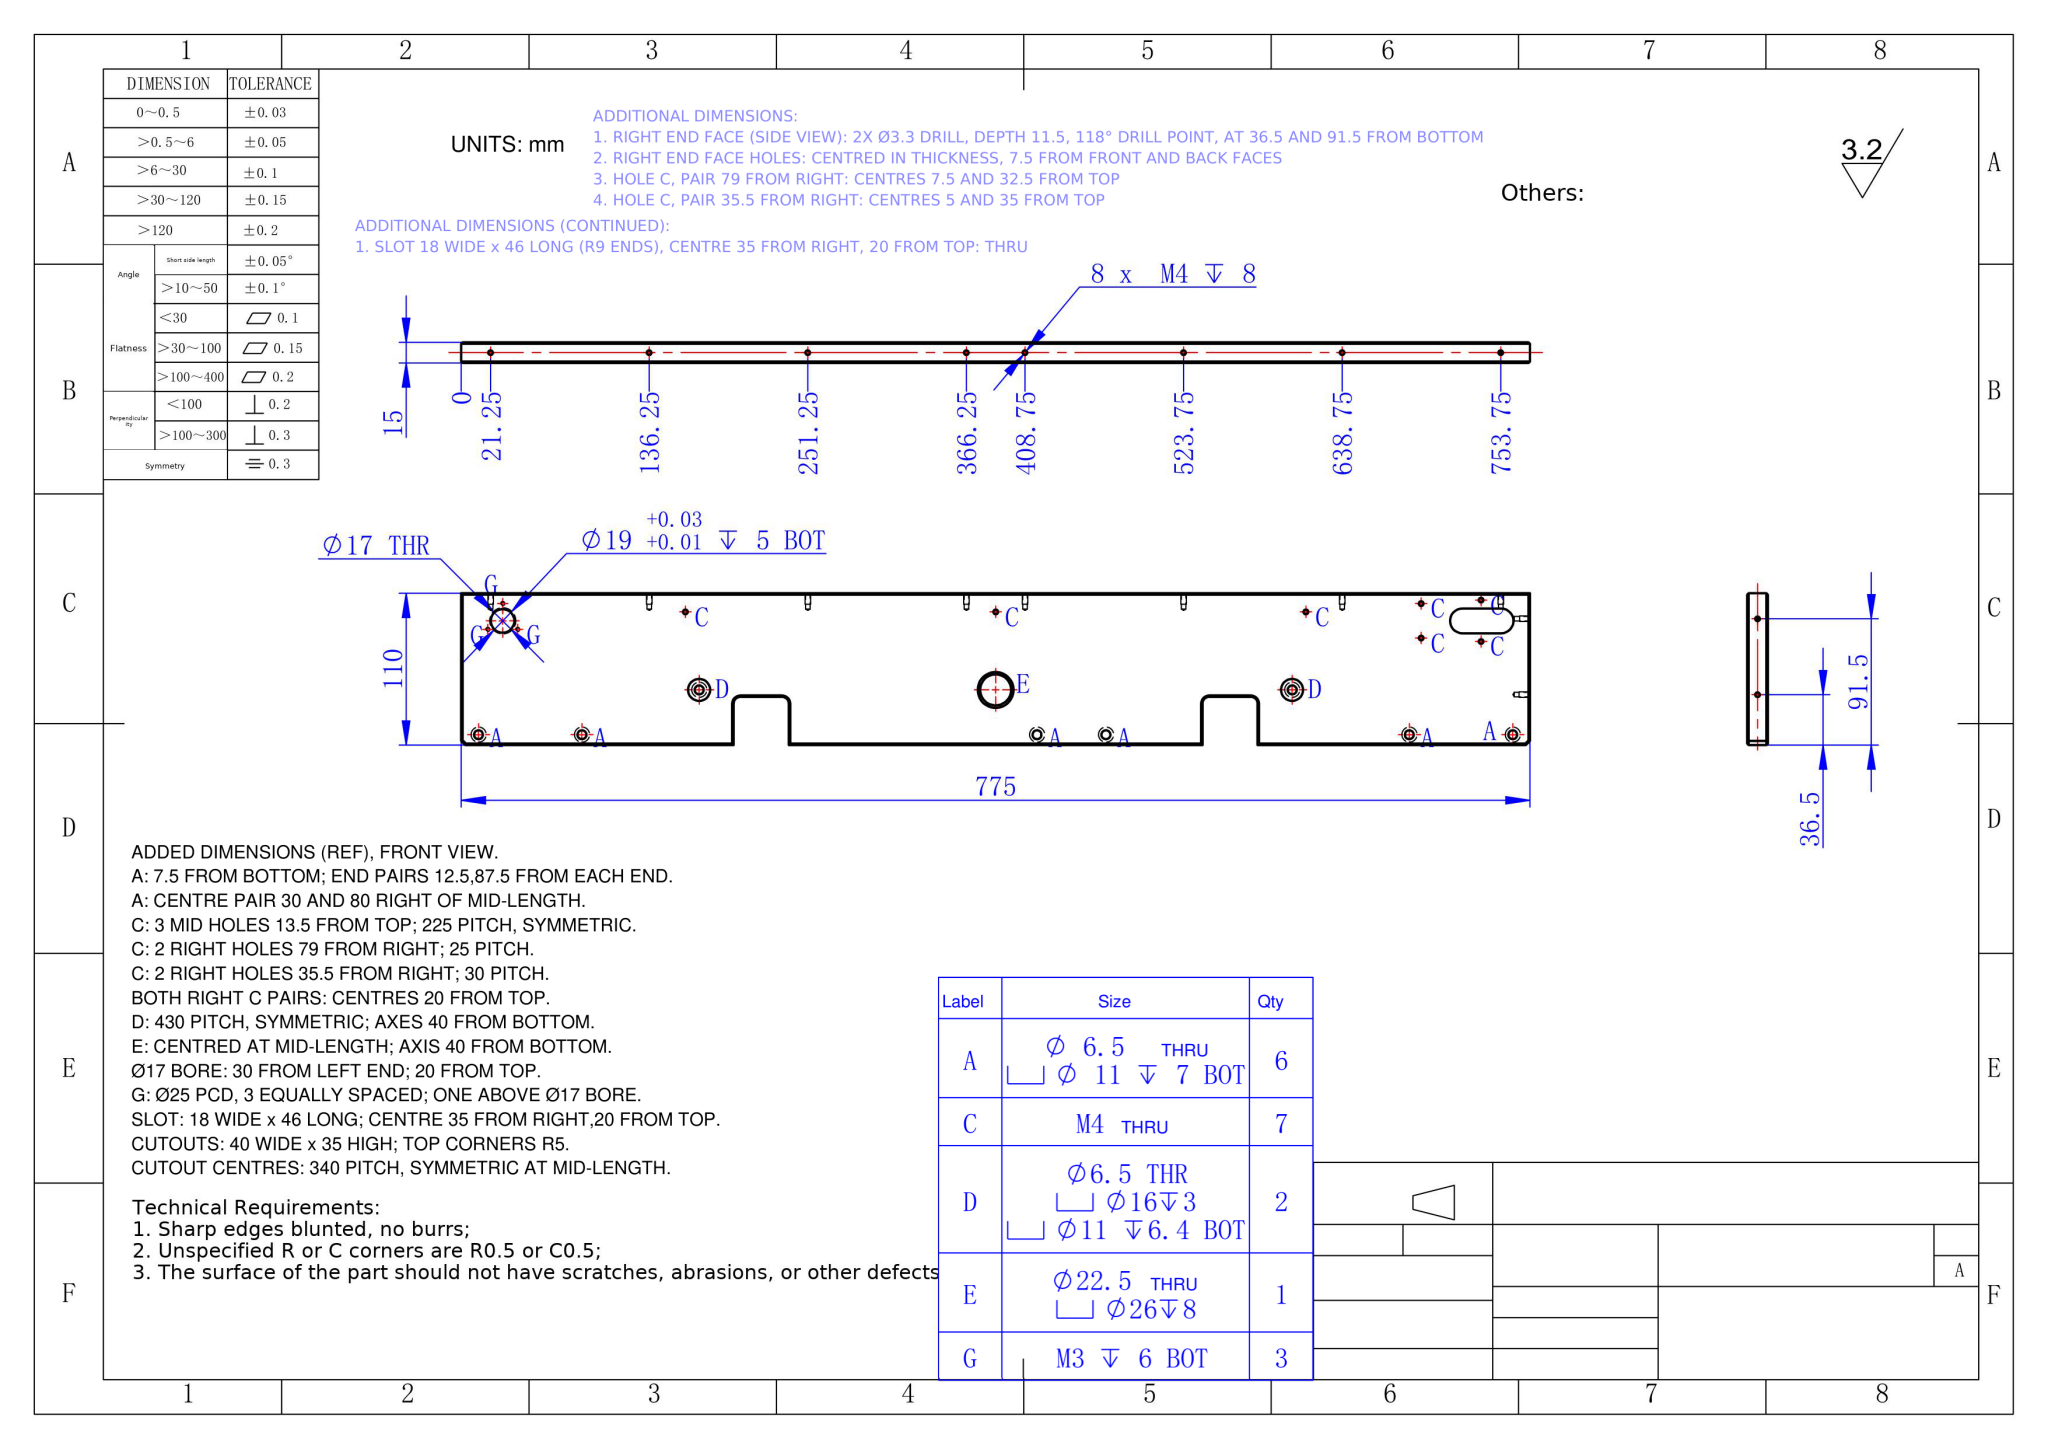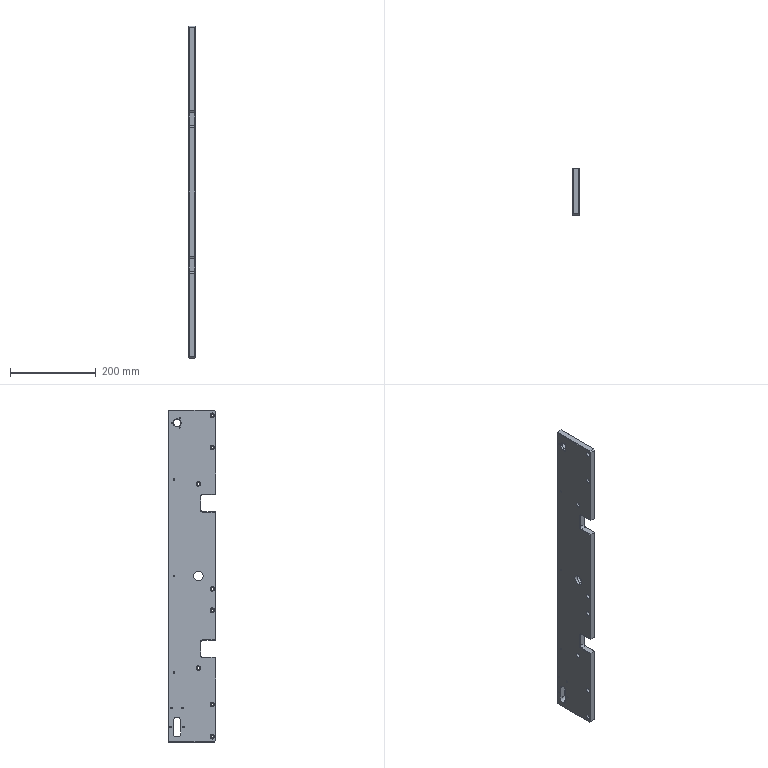Part | NX | mm | 1 solid | 181 faces | box 15 x 110 x 775 mm | volume 1202537 mm3 | cylinder 91 | plane 58 | cone 32 | commonest cylinder face diameters 3.3 x34 11 x16 6.5 x16 2.5 x6 16 x4 10 x4 18 x3 22.5 x2